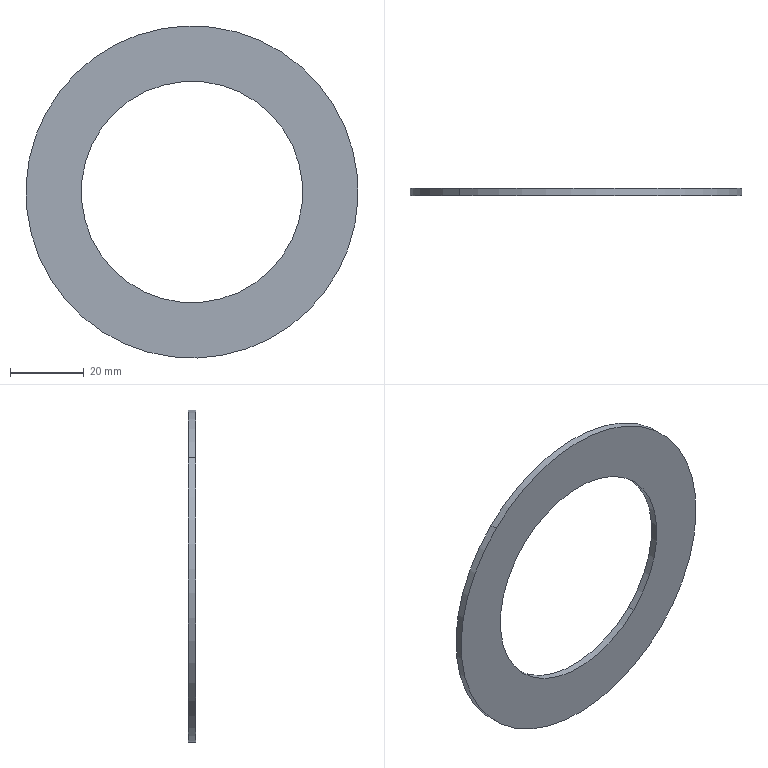Component | SolidWorks | ControlBoxGasket-1 | 1 solid | 6 faces | box 90 x 2 x 90 mm | volume 7069 mm3 | cylinder 4 | plane 2 | commonest cylinder face diameters 60 x2 90 x2
build123d program:
from build123d import *

# Parameters (mm, degrees)
SKETCH1_R           = 45
SKETCH1_R_2         = 30
BOSS_EXTRUDE1_DEPTH = 2


with BuildPart() as part:
    # Sketch1 → Boss-Extrude1 (new body)
    with BuildSketch(Plane.XY):
        Circle(SKETCH1_R)
        Circle(SKETCH1_R_2, mode=Mode.SUBTRACT)
    extrude(amount=BOSS_EXTRUDE1_DEPTH)


solid = part.part

# Placed as in the assembly
solid = solid.moved(Location((310.45, -146.434, 461.481), (90, 0, 0)))
STEP:
#1=CARTESIAN_POINT('',(11.393,-5.765,19.009));
#2=VERTEX_POINT('',#1);
#3=CARTESIAN_POINT('',(13.052,-5.765,17.328));
#4=VERTEX_POINT('',#3);
#5=CARTESIAN_POINT('',(12.222,-5.765,18.169));
#6=DIRECTION('',(-0.,1.,0.));
#7=DIRECTION('',(0.7023,0.,-0.7119));
#8=AXIS2_PLACEMENT_3D('',#5,#6,#7);
#9=CIRCLE('',#8,1.181);
#10=EDGE_CURVE('',#2,#4,#9,.T.);
#11=ORIENTED_EDGE('',*,*,#10,.T.);
#12=CARTESIAN_POINT('',(13.052,-5.844,17.328));
#13=VERTEX_POINT('',#12);
#14=CARTESIAN_POINT('',(13.052,-5.765,17.328));
#15=DIRECTION('',(0.,-1.,0.));
#16=VECTOR('',#15,39.37);
#17=LINE('',#14,#16);
#18=EDGE_CURVE('',#4,#13,#17,.T.);
#19=ORIENTED_EDGE('',*,*,#18,.T.);
#20=CARTESIAN_POINT('',(11.393,-5.844,19.009));
#21=VERTEX_POINT('',#20);
#22=CARTESIAN_POINT('',(12.222,-5.844,18.169));
#23=DIRECTION('',(-0.,1.,0.));
#24=DIRECTION('',(0.7023,0.,-0.7119));
#25=AXIS2_PLACEMENT_3D('',#22,#23,#24);
#26=CIRCLE('',#25,1.181);
#27=EDGE_CURVE('',#21,#13,#26,.T.);
#28=ORIENTED_EDGE('',*,*,#27,.F.);
#29=CARTESIAN_POINT('',(11.393,-5.765,19.009));
#30=DIRECTION('',(0.,-1.,0.));
#31=VECTOR('',#30,39.37);
#32=LINE('',#29,#31);
#33=EDGE_CURVE('',#2,#21,#32,.T.);
#34=ORIENTED_EDGE('',*,*,#33,.F.);
#35=EDGE_LOOP('',(#11,#19,#28,#34));
#36=FACE_OUTER_BOUND('',#35,.T.);
#37=CARTESIAN_POINT('',(12.222,-5.765,18.169));
#38=DIRECTION('',(0.,-1.,0.));
#39=DIRECTION('',(-0.7023,0.,0.7119));
#40=AXIS2_PLACEMENT_3D('',#37,#38,#39);
#41=CYLINDRICAL_SURFACE('',#40,1.181);
#42=ADVANCED_FACE('',(#36),#41,.F.);
#43=CARTESIAN_POINT('',(13.467,-5.765,16.907));
#44=VERTEX_POINT('',#43);
#45=CARTESIAN_POINT('',(10.978,-5.765,19.43));
#46=VERTEX_POINT('',#45);
#47=CARTESIAN_POINT('',(12.222,-5.765,18.169));
#48=DIRECTION('',(-0.,1.,0.));
#49=DIRECTION('',(0.7023,0.,-0.7119));
#50=AXIS2_PLACEMENT_3D('',#47,#48,#49);
#51=CIRCLE('',#50,1.772);
#52=EDGE_CURVE('',#44,#46,#51,.T.);
#53=ORIENTED_EDGE('',*,*,#52,.F.);
#54=CARTESIAN_POINT('',(13.467,-5.844,16.907));
#55=VERTEX_POINT('',#54);
#56=CARTESIAN_POINT('',(13.467,-5.765,16.907));
#57=DIRECTION('',(0.,-1.,0.));
#58=VECTOR('',#57,39.37);
#59=LINE('',#56,#58);
#60=EDGE_CURVE('',#44,#55,#59,.T.);
#61=ORIENTED_EDGE('',*,*,#60,.T.);
#62=CARTESIAN_POINT('',(10.978,-5.844,19.43));
#63=VERTEX_POINT('',#62);
#64=CARTESIAN_POINT('',(12.222,-5.844,18.169));
#65=DIRECTION('',(-0.,1.,0.));
#66=DIRECTION('',(0.7023,0.,-0.7119));
#67=AXIS2_PLACEMENT_3D('',#64,#65,#66);
#68=CIRCLE('',#67,1.772);
#69=EDGE_CURVE('',#55,#63,#68,.T.);
#70=ORIENTED_EDGE('',*,*,#69,.T.);
#71=CARTESIAN_POINT('',(10.978,-5.765,19.43));
#72=DIRECTION('',(0.,-1.,0.));
#73=VECTOR('',#72,39.37);
#74=LINE('',#71,#73);
#75=EDGE_CURVE('',#46,#63,#74,.T.);
#76=ORIENTED_EDGE('',*,*,#75,.F.);
#77=EDGE_LOOP('',(#53,#61,#70,#76));
#78=FACE_OUTER_BOUND('',#77,.T.);
#79=CARTESIAN_POINT('',(12.222,-5.765,18.169));
#80=DIRECTION('',(0.,-1.,0.));
#81=DIRECTION('',(-0.7023,0.,0.7119));
#82=AXIS2_PLACEMENT_3D('',#79,#80,#81);
#83=CYLINDRICAL_SURFACE('',#82,1.772);
#84=ADVANCED_FACE('',(#78),#83,.T.);
#85=CARTESIAN_POINT('',(12.222,-5.765,18.169));
#86=DIRECTION('',(-0.,1.,0.));
#87=DIRECTION('',(0.7023,0.,-0.7119));
#88=AXIS2_PLACEMENT_3D('',#85,#86,#87);
#89=CIRCLE('',#88,1.772);
#90=EDGE_CURVE('',#46,#44,#89,.T.);
#91=ORIENTED_EDGE('',*,*,#90,.T.);
#92=ORIENTED_EDGE('',*,*,#52,.T.);
#93=EDGE_LOOP('',(#91,#92));
#94=FACE_OUTER_BOUND('',#93,.T.);
#95=ORIENTED_EDGE('',*,*,#10,.F.);
#96=CARTESIAN_POINT('',(12.222,-5.765,18.169));
#97=DIRECTION('',(-0.,1.,0.));
#98=DIRECTION('',(0.7023,0.,-0.7119));
#99=AXIS2_PLACEMENT_3D('',#96,#97,#98);
#100=CIRCLE('',#99,1.181);
#101=EDGE_CURVE('',#4,#2,#100,.T.);
#102=ORIENTED_EDGE('',*,*,#101,.F.);
#103=EDGE_LOOP('',(#95,#102));
#104=FACE_BOUND('',#103,.T.);
#105=CARTESIAN_POINT('',(12.222,-5.765,18.169));
#106=DIRECTION('',(-0.,1.,-0.));
#107=DIRECTION('',(0.7023,0.,-0.7119));
#108=AXIS2_PLACEMENT_3D('',#105,#106,#107);
#109=PLANE('',#108);
#110=ADVANCED_FACE('',(#94,#104),#109,.T.);
#111=CARTESIAN_POINT('',(12.222,-5.844,18.169));
#112=DIRECTION('',(-0.,1.,0.));
#113=DIRECTION('',(0.7023,0.,-0.7119));
#114=AXIS2_PLACEMENT_3D('',#111,#112,#113);
#115=CIRCLE('',#114,1.772);
#116=EDGE_CURVE('',#63,#55,#115,.T.);
#117=ORIENTED_EDGE('',*,*,#116,.F.);
#118=ORIENTED_EDGE('',*,*,#69,.F.);
#119=EDGE_LOOP('',(#117,#118));
#120=FACE_OUTER_BOUND('',#119,.T.);
#121=ORIENTED_EDGE('',*,*,#27,.T.);
#122=CARTESIAN_POINT('',(12.222,-5.844,18.169));
#123=DIRECTION('',(-0.,1.,0.));
#124=DIRECTION('',(0.7023,0.,-0.7119));
#125=AXIS2_PLACEMENT_3D('',#122,#123,#124);
#126=CIRCLE('',#125,1.181);
#127=EDGE_CURVE('',#13,#21,#126,.T.);
#128=ORIENTED_EDGE('',*,*,#127,.T.);
#129=EDGE_LOOP('',(#121,#128));
#130=FACE_BOUND('',#129,.T.);
#131=CARTESIAN_POINT('',(12.222,-5.844,18.169));
#132=DIRECTION('',(-0.,1.,-0.));
#133=DIRECTION('',(0.7023,0.,-0.7119));
#134=AXIS2_PLACEMENT_3D('',#131,#132,#133);
#135=PLANE('',#134);
#136=ADVANCED_FACE('',(#120,#130),#135,.F.);
#137=ORIENTED_EDGE('',*,*,#60,.F.);
#138=ORIENTED_EDGE('',*,*,#90,.F.);
#139=ORIENTED_EDGE('',*,*,#75,.T.);
#140=ORIENTED_EDGE('',*,*,#116,.T.);
#141=EDGE_LOOP('',(#137,#138,#139,#140));
#142=FACE_OUTER_BOUND('',#141,.T.);
#143=CARTESIAN_POINT('',(12.222,-5.765,18.169));
#144=DIRECTION('',(0.,-1.,0.));
#145=DIRECTION('',(-0.7023,0.,0.7119));
#146=AXIS2_PLACEMENT_3D('',#143,#144,#145);
#147=CYLINDRICAL_SURFACE('',#146,1.772);
#148=ADVANCED_FACE('',(#142),#147,.T.);
#149=ORIENTED_EDGE('',*,*,#18,.F.);
#150=ORIENTED_EDGE('',*,*,#101,.T.);
#151=ORIENTED_EDGE('',*,*,#33,.T.);
#152=ORIENTED_EDGE('',*,*,#127,.F.);
#153=EDGE_LOOP('',(#149,#150,#151,#152));
#154=FACE_OUTER_BOUND('',#153,.T.);
#155=CARTESIAN_POINT('',(12.222,-5.765,18.169));
#156=DIRECTION('',(0.,-1.,0.));
#157=DIRECTION('',(-0.7023,0.,0.7119));
#158=AXIS2_PLACEMENT_3D('',#155,#156,#157);
#159=CYLINDRICAL_SURFACE('',#158,1.181);
#160=ADVANCED_FACE('',(#154),#159,.F.);
#161=CLOSED_SHELL('',(#42,#84,#110,#136,#148,#160));
#162=MANIFOLD_SOLID_BREP('',#161);
#163=CARTESIAN_POINT('',(0.,0.,0.));
#164=DIRECTION('',(0.,0.,1.));
#165=DIRECTION('',(1.,0.,0.));
#166=AXIS2_PLACEMENT_3D('',#163,#164,#165);
#167=(LENGTH_UNIT()NAMED_UNIT(*)SI_UNIT($,.METRE.));
#168=LENGTH_MEASURE_WITH_UNIT(LENGTH_MEASURE(0.0254),#167);
#169=DIMENSIONAL_EXPONENTS(1.,0.,0.,0.,0.,0.,0.);
#170=(CONVERSION_BASED_UNIT('',#168)LENGTH_UNIT()NAMED_UNIT(#169));
#171=UNCERTAINTY_MEASURE_WITH_UNIT(LENGTH_MEASURE(0.00001),#170,'','');
#172=(NAMED_UNIT(*)PLANE_ANGLE_UNIT()SI_UNIT($,.RADIAN.));
#173=(NAMED_UNIT(*)SI_UNIT($,.STERADIAN.)SOLID_ANGLE_UNIT());
#174=(GEOMETRIC_REPRESENTATION_CONTEXT(3)GLOBAL_UNCERTAINTY_ASSIGNED_CONTEXT((#171))GLOBAL_UNIT_ASSIGNED_CONTEXT((#170,#172,#173))REPRESENTATION_CONTEXT('',''));
#175=ADVANCED_BREP_SHAPE_REPRESENTATION('',(#162,#166),#174);
#176=COLOUR_RGB('',0.7922,0.8196,0.9333);
#177=FILL_AREA_STYLE_COLOUR('',#176);
#178=FILL_AREA_STYLE('',(#177));
#179=SURFACE_STYLE_FILL_AREA(#178);
#180=SURFACE_SIDE_STYLE('',(#179));
#181=SURFACE_STYLE_USAGE(.BOTH.,#180);
#182=PRESENTATION_STYLE_ASSIGNMENT((#181));
#183=STYLED_ITEM('',(#182),#162);
#184=(LENGTH_UNIT()NAMED_UNIT(*)SI_UNIT($,.METRE.));
#185=LENGTH_MEASURE_WITH_UNIT(LENGTH_MEASURE(0.0254),#184);
#186=DIMENSIONAL_EXPONENTS(1.,0.,0.,0.,0.,0.,0.);
#187=(CONVERSION_BASED_UNIT('',#185)LENGTH_UNIT()NAMED_UNIT(#186));
#188=UNCERTAINTY_MEASURE_WITH_UNIT(LENGTH_MEASURE(0.00001),#187,'','');
#189=(NAMED_UNIT(*)PLANE_ANGLE_UNIT()SI_UNIT($,.RADIAN.));
#190=(NAMED_UNIT(*)SI_UNIT($,.STERADIAN.)SOLID_ANGLE_UNIT());
#191=(GEOMETRIC_REPRESENTATION_CONTEXT(3)GLOBAL_UNCERTAINTY_ASSIGNED_CONTEXT((#188))GLOBAL_UNIT_ASSIGNED_CONTEXT((#187,#189,#190))REPRESENTATION_CONTEXT('',''));
#192=MECHANICAL_DESIGN_GEOMETRIC_PRESENTATION_REPRESENTATION('',(#183),#191);
#193=PRESENTATION_LAYER_ASSIGNMENT('','',(#183));